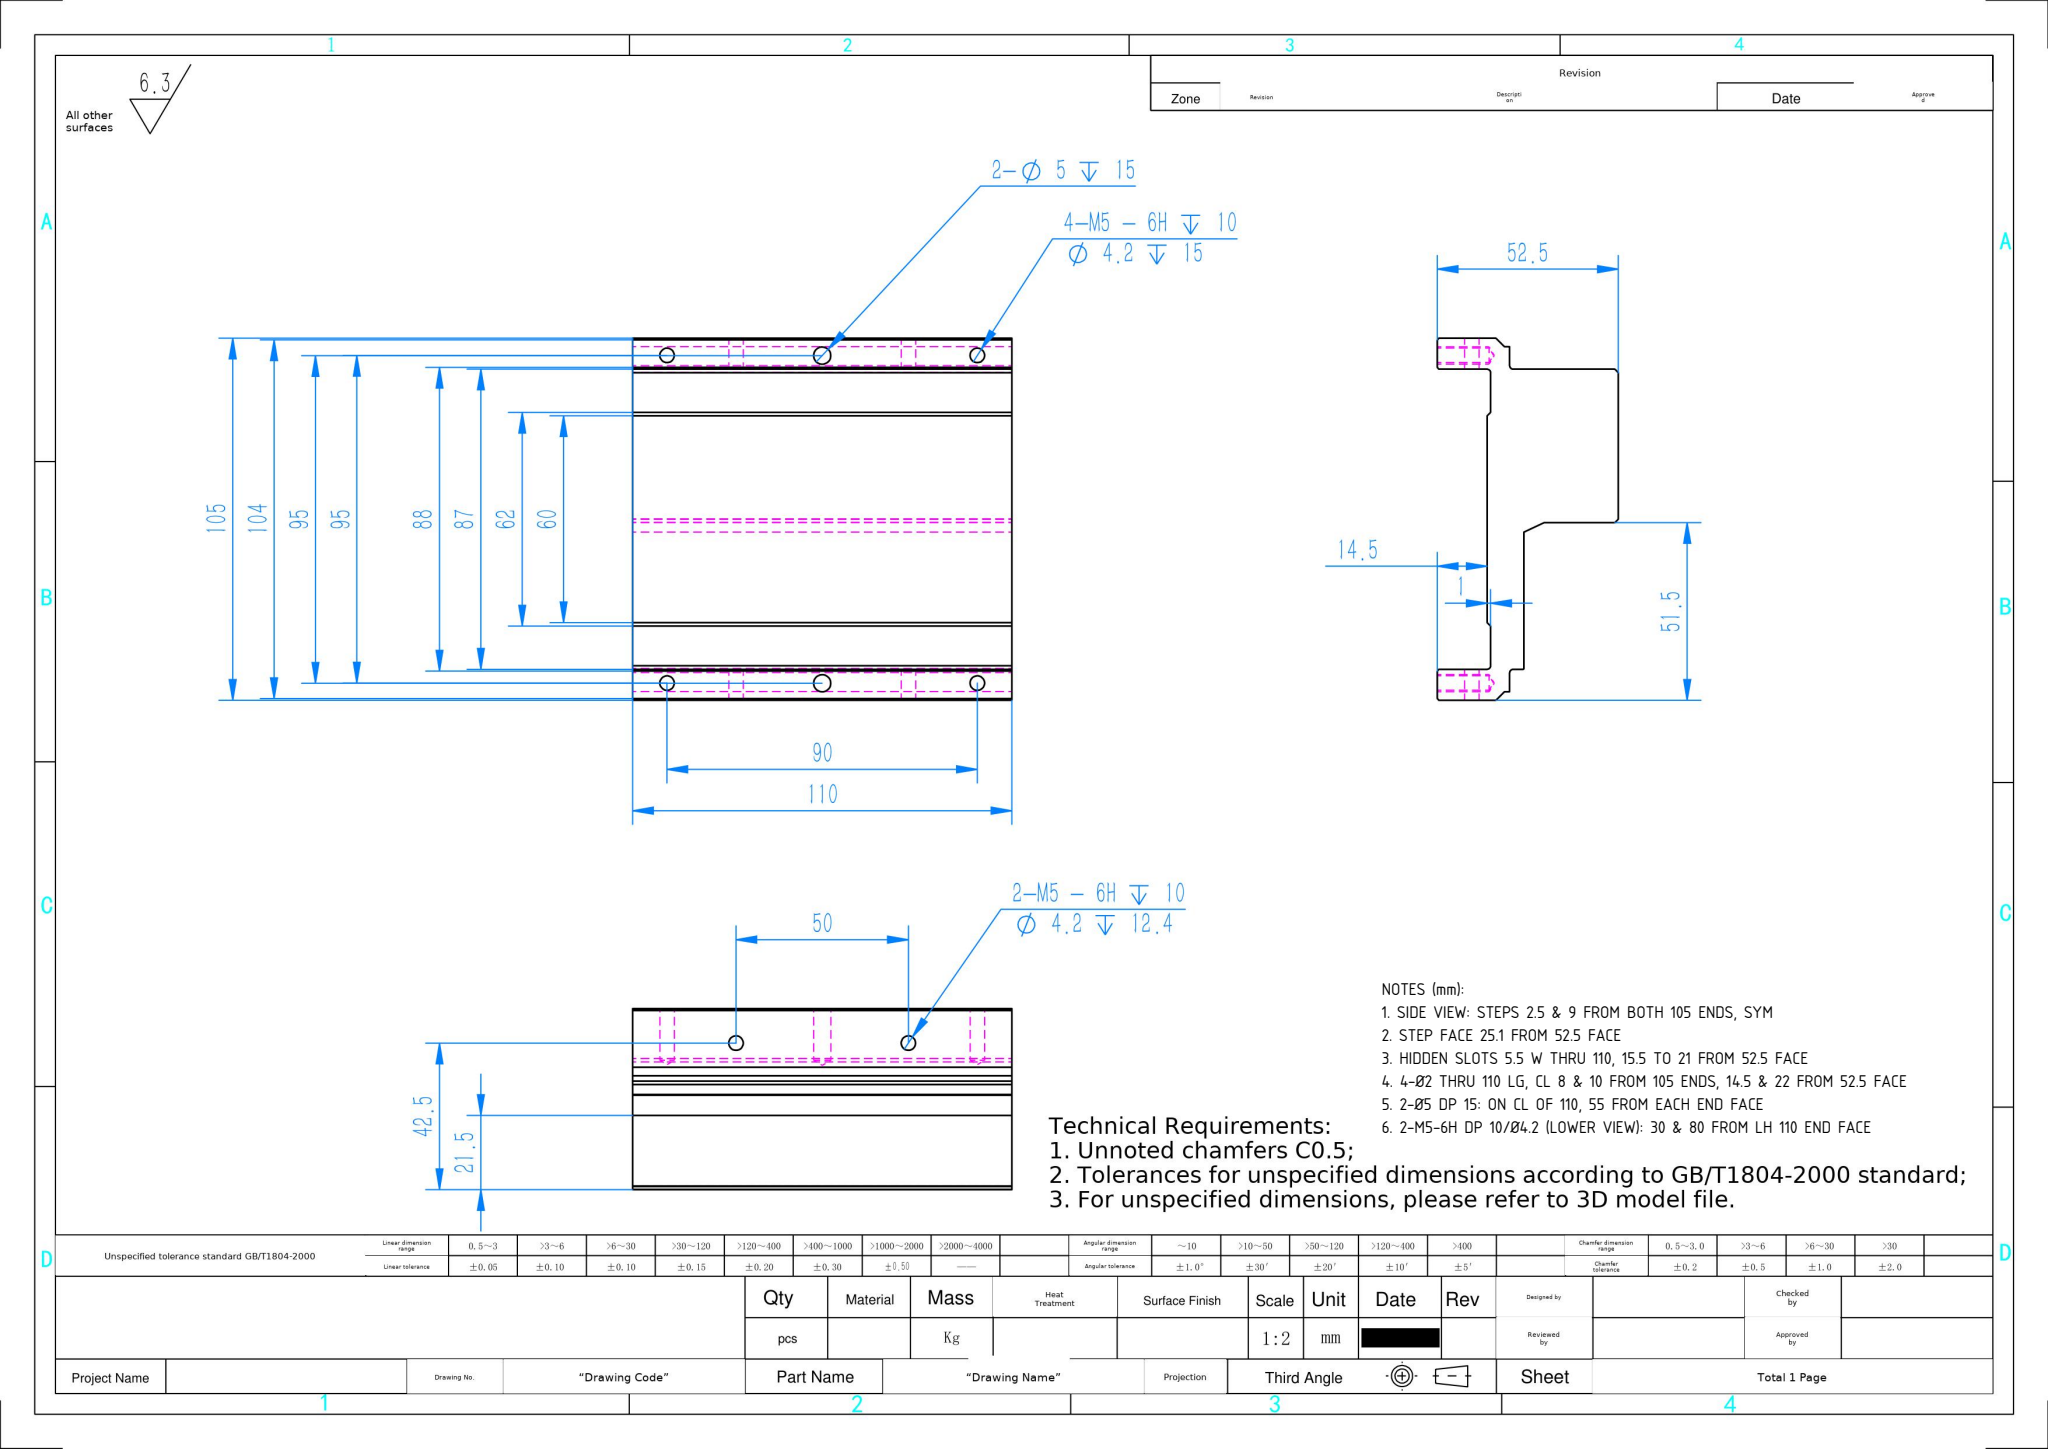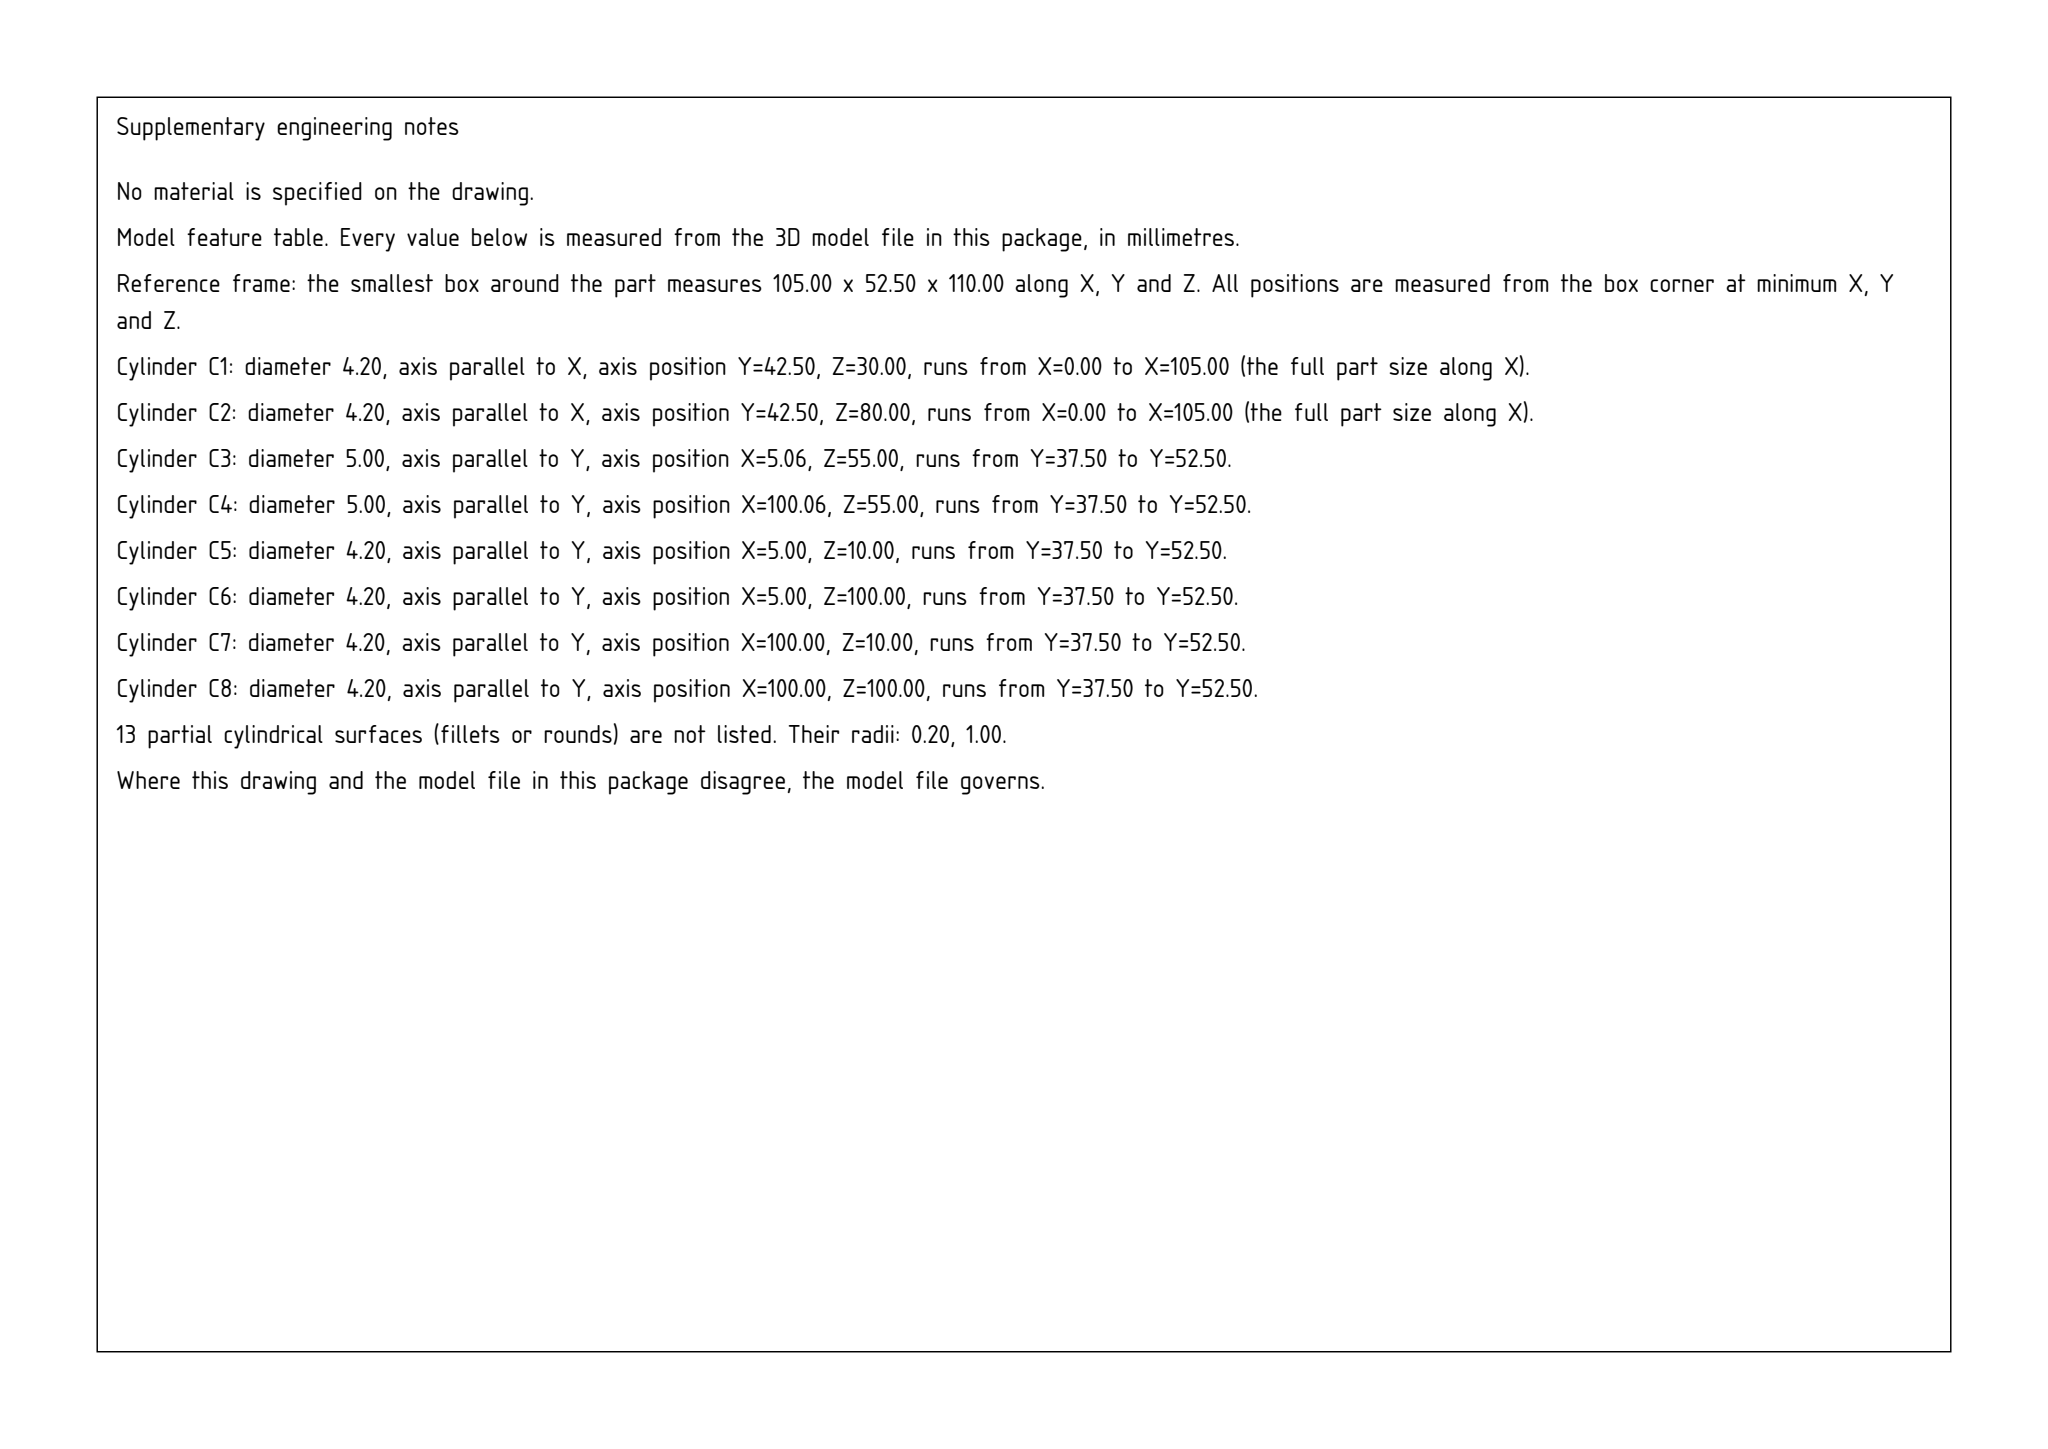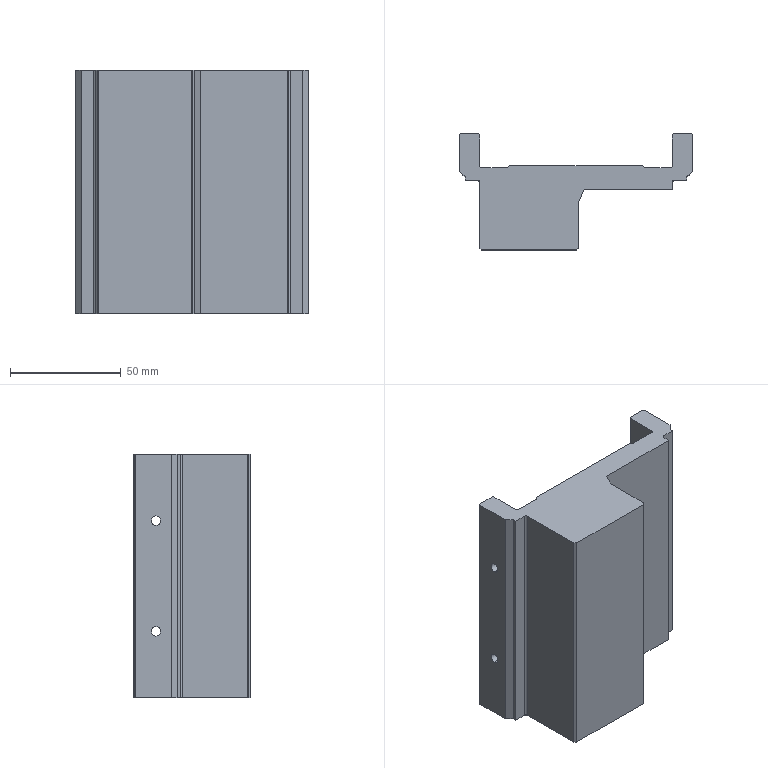Part | SolidWorks | mm | 1 solid | 76 faces | box 105 x 52.5 x 110 mm | volume 271636 mm3 | cylinder 33 | plane 31 | cone 12 | commonest cylinder face diameters 4.2 x16 0.4 x9 5 x4 2 x4
Drawing notes:
SIDE VIEW: STEPS 2.5 & 9 FROM BOTH 105 ENDS, SYM | from the solid: x-planes 2.5, 9.0 and 96.0, 102.5 in bbox x=0..105 (symmetric)
STEP FACE 25.1 FROM 52.5 FACE | from the solid: y-plane 27.4 vs y=52.5 outer face (52.5-27.4=25.1)
HIDDEN SLOTS 5.5 W THRU 110, 15.5 TO 21 FROM 52.5 FACE | from the solid: paired y-planes 37.0 & 31.5 (5.5 apart), run full z=0..110; 52.5-37=15.5, 52.5-31.5=21
4-Ø2 THRU 110 LG, CL 8 & 10 FROM 105 ENDS, 14.5 & 22 FROM 52.5 FACE | from the solid: Ø2 cyls axis z at x=8.0, 10.0, 95.0, 97.0, len 110; y=38.0 & 30.5 (52.5-38=14.5, 52.5-30.5=22)
2-Ø5 DP 15: ON CL OF 110, 55 FROM EACH END FACE | from the solid: Ø5 y-axis holes at z=55.0 (x=5.06 & 100.06), bbox z=110
2-M5-6H DP 10/Ø4.2 (LOWER VIEW): 30 & 80 FROM LH 110 END FACE | from the solid: Ø4.2 x-axis holes at z=30.0 and z=80.0, y=42.5, bbox z=110